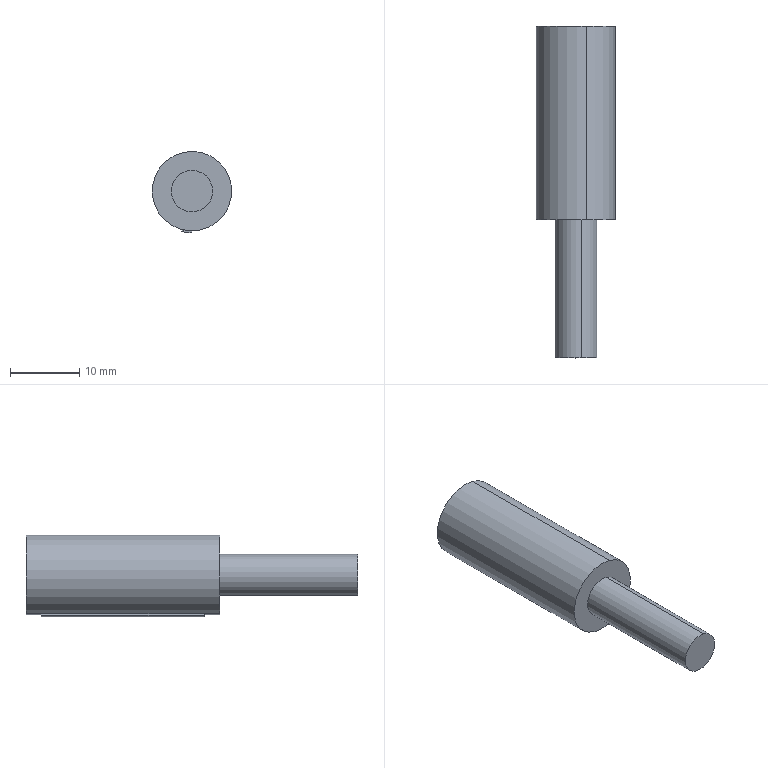Component | SolidWorks | Hinge2-1 | 1 solid | 13 faces | box 11.5 x 48 x 11.75 mm | volume 3483 mm3 | plane 9 | cylinder 4 | commonest cylinder face diameters 6 x2 11.5 x2
build123d program:
from build123d import *

# Parameters (mm, degrees)
SKETCH1_2_R              = 5.75
BOSS_EXTRUDE1_DEPTH      = 14
BOSS_EXTRUDE2_REACH      = 23.728
BOSS_EXTRUDE2_END_RADIUS = 5.75
SKETCH2_W                = 1.461
SKETCH2_H                = 23.562
SKETCH3_R                = 3
BOSS_EXTRUDE3_DEPTH      = 20
CUT_EXTRUDE1_DEPTH       = 13
CUT_EXTRUDE1_DEPTH_BACK  = 13


with BuildPart() as part:
    # Sketch1_2 → Boss-Extrude1 (new, symmetric)
    with BuildSketch(Plane(origin=(0, 0, 0), x_dir=(1, 0, 0), z_dir=(0, 1, 0))):
        with Locations(Location((-6, -6, 0), (0, 0, 270))):
            Circle(SKETCH1_2_R)
    extrude(amount=BOSS_EXTRUDE1_DEPTH, both=True)

    # Boss-Extrude2: up to this cylinder (the profile starts outside it)
    boss_extrude2_end = Plane(origin=(-6, 0, 6), z_dir=(0, -1, 0)) * Cylinder(BOSS_EXTRUDE2_END_RADIUS, 59.956, mode=Mode.PRIVATE)
    # Sketch2 → Boss-Extrude2 (add, up to the surface)
    with BuildSketch(Plane.XY, mode=Mode.PRIVATE) as boss_extrude2_sk1:
        with Locations((-5.269, 0)):
            Rectangle(SKETCH2_W, SKETCH2_H)
    boss_extrude2_tool1 = extrude(boss_extrude2_sk1.sketch, amount=BOSS_EXTRUDE2_REACH, mode=Mode.PRIVATE) - boss_extrude2_end
    add(boss_extrude2_tool1.solids().sort_by_distance((-5.269, 0, 0))[0])

    # Sketch3 → Boss-Extrude3 (add)
    with BuildSketch(Plane.XZ.offset(14)):
        with Locations(Location((-6, 6, 0), (0, 0, 90))):
            Circle(SKETCH3_R)
    extrude(amount=BOSS_EXTRUDE3_DEPTH)

    # Sketch1 → Cut-Extrude1 (cut, two sides: drawn at the far end of the back side and taken through both)
    with BuildSketch(Plane(origin=(0, 0, 0), x_dir=(1, 0, 0), z_dir=(0, 1, 0)).offset(-CUT_EXTRUDE1_DEPTH_BACK)):
        Polygon((-7.5, 0.6087), (-3, -0.5914), (-3, 2), (-7.5, 2), align=None)
    extrude(amount=CUT_EXTRUDE1_DEPTH + CUT_EXTRUDE1_DEPTH_BACK, mode=Mode.SUBTRACT)


solid = part.part

# Placed as in the assembly
solid = solid.moved(Location((227.642, -308.131, 905.044), (0, 14.933, 0)))
STEP:
#1=CARTESIAN_POINT('',(8.764,-13.47,35.807));
#2=VERTEX_POINT('',#1);
#3=CARTESIAN_POINT('',(8.825,-13.47,36.035));
#4=VERTEX_POINT('',#3);
#5=CARTESIAN_POINT('',(8.795,-13.47,35.921));
#6=DIRECTION('',(0.,-1.,0.));
#7=DIRECTION('',(-0.2577,0.,-0.9662));
#8=AXIS2_PLACEMENT_3D('',#5,#6,#7);
#9=CIRCLE('',#8,0.1181);
#10=EDGE_CURVE('',#2,#4,#9,.T.);
#11=ORIENTED_EDGE('',*,*,#10,.F.);
#12=CARTESIAN_POINT('',(8.764,-12.682,35.807));
#13=VERTEX_POINT('',#12);
#14=CARTESIAN_POINT('',(8.764,-13.47,35.807));
#15=DIRECTION('',(0.,1.,0.));
#16=VECTOR('',#15,39.37);
#17=LINE('',#14,#16);
#18=EDGE_CURVE('',#2,#13,#17,.T.);
#19=ORIENTED_EDGE('',*,*,#18,.T.);
#20=CARTESIAN_POINT('',(8.825,-12.682,36.035));
#21=VERTEX_POINT('',#20);
#22=CARTESIAN_POINT('',(8.795,-12.682,35.921));
#23=DIRECTION('',(0.,-1.,0.));
#24=DIRECTION('',(0.2577,0.,0.9662));
#25=AXIS2_PLACEMENT_3D('',#22,#23,#24);
#26=CIRCLE('',#25,0.1181);
#27=EDGE_CURVE('',#13,#21,#26,.T.);
#28=ORIENTED_EDGE('',*,*,#27,.T.);
#29=CARTESIAN_POINT('',(8.825,-13.47,36.035));
#30=DIRECTION('',(0.,1.,0.));
#31=VECTOR('',#30,39.37);
#32=LINE('',#29,#31);
#33=EDGE_CURVE('',#4,#21,#32,.T.);
#34=ORIENTED_EDGE('',*,*,#33,.F.);
#35=EDGE_LOOP('',(#11,#19,#28,#34));
#36=FACE_OUTER_BOUND('',#35,.T.);
#37=CARTESIAN_POINT('',(8.795,-13.47,35.921));
#38=DIRECTION('',(0.,1.,0.));
#39=DIRECTION('',(0.2577,0.,0.9662));
#40=AXIS2_PLACEMENT_3D('',#37,#38,#39);
#41=CYLINDRICAL_SURFACE('',#40,0.1181);
#42=ADVANCED_FACE('',(#36),#41,.T.);
#43=CARTESIAN_POINT('',(8.853,-11.58,36.139));
#44=VERTEX_POINT('',#43);
#45=CARTESIAN_POINT('',(8.737,-11.58,35.702));
#46=VERTEX_POINT('',#45);
#47=CARTESIAN_POINT('',(8.795,-11.58,35.921));
#48=DIRECTION('',(0.,1.,0.));
#49=DIRECTION('',(0.2577,0.,0.9662));
#50=AXIS2_PLACEMENT_3D('',#47,#48,#49);
#51=CIRCLE('',#50,0.2264);
#52=EDGE_CURVE('',#44,#46,#51,.T.);
#53=ORIENTED_EDGE('',*,*,#52,.F.);
#54=CARTESIAN_POINT('',(8.853,-12.682,36.139));
#55=VERTEX_POINT('',#54);
#56=CARTESIAN_POINT('',(8.853,-11.58,36.139));
#57=DIRECTION('',(0.,-1.,0.));
#58=VECTOR('',#57,39.37);
#59=LINE('',#56,#58);
#60=EDGE_CURVE('',#44,#55,#59,.T.);
#61=ORIENTED_EDGE('',*,*,#60,.T.);
#62=CARTESIAN_POINT('',(8.737,-12.682,35.702));
#63=VERTEX_POINT('',#62);
#64=CARTESIAN_POINT('',(8.795,-12.682,35.921));
#65=DIRECTION('',(0.,1.,0.));
#66=DIRECTION('',(0.2577,0.,0.9662));
#67=AXIS2_PLACEMENT_3D('',#64,#65,#66);
#68=CIRCLE('',#67,0.2264);
#69=EDGE_CURVE('',#55,#63,#68,.T.);
#70=ORIENTED_EDGE('',*,*,#69,.T.);
#71=CARTESIAN_POINT('',(8.737,-12.595,35.702));
#72=VERTEX_POINT('',#71);
#73=CARTESIAN_POINT('',(8.737,-11.58,35.702));
#74=DIRECTION('',(0.,-1.,0.));
#75=VECTOR('',#74,39.37);
#76=LINE('',#73,#75);
#77=EDGE_CURVE('',#72,#63,#76,.T.);
#78=ORIENTED_EDGE('',*,*,#77,.F.);
#79=CARTESIAN_POINT('',(8.794,-12.595,35.694));
#80=VERTEX_POINT('',#79);
#81=CARTESIAN_POINT('',(8.795,-12.595,35.921));
#82=DIRECTION('',(0.,-1.,0.));
#83=DIRECTION('',(0.2577,0.,0.9662));
#84=AXIS2_PLACEMENT_3D('',#81,#82,#83);
#85=CIRCLE('',#84,0.2264);
#86=EDGE_CURVE('',#72,#80,#85,.T.);
#87=ORIENTED_EDGE('',*,*,#86,.T.);
#88=CARTESIAN_POINT('',(8.794,-11.667,35.694));
#89=VERTEX_POINT('',#88);
#90=CARTESIAN_POINT('',(8.794,-11.58,35.694));
#91=DIRECTION('',(0.,1.,0.));
#92=VECTOR('',#91,39.37);
#93=LINE('',#90,#92);
#94=EDGE_CURVE('',#80,#89,#93,.T.);
#95=ORIENTED_EDGE('',*,*,#94,.T.);
#96=CARTESIAN_POINT('',(8.737,-11.667,35.702));
#97=VERTEX_POINT('',#96);
#98=CARTESIAN_POINT('',(8.795,-11.667,35.921));
#99=DIRECTION('',(0.,1.,0.));
#100=DIRECTION('',(-0.2577,0.,-0.9662));
#101=AXIS2_PLACEMENT_3D('',#98,#99,#100);
#102=CIRCLE('',#101,0.2264);
#103=EDGE_CURVE('',#89,#97,#102,.T.);
#104=ORIENTED_EDGE('',*,*,#103,.T.);
#105=CARTESIAN_POINT('',(8.737,-11.58,35.702));
#106=DIRECTION('',(0.,-1.,0.));
#107=VECTOR('',#106,39.37);
#108=LINE('',#105,#107);
#109=EDGE_CURVE('',#46,#97,#108,.T.);
#110=ORIENTED_EDGE('',*,*,#109,.F.);
#111=EDGE_LOOP('',(#53,#61,#70,#78,#87,#95,#104,#110));
#112=FACE_OUTER_BOUND('',#111,.T.);
#113=CARTESIAN_POINT('',(8.795,-11.58,35.921));
#114=DIRECTION('',(0.,-1.,0.));
#115=DIRECTION('',(-0.2577,0.,-0.9662));
#116=AXIS2_PLACEMENT_3D('',#113,#114,#115);
#117=CYLINDRICAL_SURFACE('',#116,0.2264);
#118=ADVANCED_FACE('',(#112),#117,.T.);
#119=CARTESIAN_POINT('',(8.791,-12.595,35.685));
#120=VERTEX_POINT('',#119);
#121=CARTESIAN_POINT('',(8.764,-12.595,35.685));
#122=VERTEX_POINT('',#121);
#123=CARTESIAN_POINT('',(5081.383,-12.595,35.685));
#124=DIRECTION('',(-1.,0.,-0.));
#125=VECTOR('',#124,39.37);
#126=LINE('',#123,#125);
#127=EDGE_CURVE('',#120,#122,#126,.T.);
#128=ORIENTED_EDGE('',*,*,#127,.F.);
#129=CARTESIAN_POINT('',(5081.383,-12.595,19055.919));
#130=DIRECTION('',(-0.2577,0.,-0.9662));
#131=VECTOR('',#130,39.37);
#132=LINE('',#129,#131);
#133=EDGE_CURVE('',#80,#120,#132,.T.);
#134=ORIENTED_EDGE('',*,*,#133,.F.);
#135=ORIENTED_EDGE('',*,*,#86,.F.);
#136=CARTESIAN_POINT('',(8.734,-12.595,35.693));
#137=VERTEX_POINT('',#136);
#138=CARTESIAN_POINT('',(5081.327,-12.595,19055.934));
#139=DIRECTION('',(-0.2577,0.,-0.9662));
#140=VECTOR('',#139,39.37);
#141=LINE('',#138,#140);
#142=EDGE_CURVE('',#72,#137,#141,.T.);
#143=ORIENTED_EDGE('',*,*,#142,.T.);
#144=CARTESIAN_POINT('',(8.79,-12.595,35.678));
#145=DIRECTION('',(0.9662,0.,-0.2577));
#146=VECTOR('',#145,39.37);
#147=LINE('',#144,#146);
#148=EDGE_CURVE('',#137,#122,#147,.T.);
#149=ORIENTED_EDGE('',*,*,#148,.T.);
#150=EDGE_LOOP('',(#128,#134,#135,#143,#149));
#151=FACE_OUTER_BOUND('',#150,.T.);
#152=CARTESIAN_POINT('',(5081.383,-12.595,19055.919));
#153=DIRECTION('',(0.,1.,0.));
#154=DIRECTION('',(0.2577,0.,0.9662));
#155=AXIS2_PLACEMENT_3D('',#152,#153,#154);
#156=PLANE('',#155);
#157=ADVANCED_FACE('',(#151),#156,.F.);
#158=CARTESIAN_POINT('',(8.764,-11.667,35.685));
#159=VERTEX_POINT('',#158);
#160=CARTESIAN_POINT('',(8.764,-12.131,35.685));
#161=DIRECTION('',(0.,1.,0.));
#162=VECTOR('',#161,39.37);
#163=LINE('',#160,#162);
#164=EDGE_CURVE('',#122,#159,#163,.T.);
#165=ORIENTED_EDGE('',*,*,#164,.F.);
#166=ORIENTED_EDGE('',*,*,#148,.F.);
#167=CARTESIAN_POINT('',(8.734,-11.667,35.693));
#168=VERTEX_POINT('',#167);
#169=CARTESIAN_POINT('',(8.734,-12.595,35.693));
#170=DIRECTION('',(0.,-1.,0.));
#171=VECTOR('',#170,39.37);
#172=LINE('',#169,#171);
#173=EDGE_CURVE('',#168,#137,#172,.T.);
#174=ORIENTED_EDGE('',*,*,#173,.F.);
#175=CARTESIAN_POINT('',(8.79,-11.667,35.678));
#176=DIRECTION('',(-0.9662,0.,0.2577));
#177=VECTOR('',#176,39.37);
#178=LINE('',#175,#177);
#179=EDGE_CURVE('',#159,#168,#178,.T.);
#180=ORIENTED_EDGE('',*,*,#179,.F.);
#181=EDGE_LOOP('',(#165,#166,#174,#180));
#182=FACE_OUTER_BOUND('',#181,.T.);
#183=CARTESIAN_POINT('',(8.962,-12.131,35.632));
#184=DIRECTION('',(0.2577,0.,0.9662));
#185=DIRECTION('',(0.9662,0.,-0.2577));
#186=AXIS2_PLACEMENT_3D('',#183,#184,#185);
#187=PLANE('',#186);
#188=ADVANCED_FACE('',(#182),#187,.F.);
#189=CARTESIAN_POINT('',(8.791,-11.667,35.685));
#190=VERTEX_POINT('',#189);
#191=CARTESIAN_POINT('',(8.791,-12.595,35.685));
#192=DIRECTION('',(0.,-1.,0.));
#193=VECTOR('',#192,39.37);
#194=LINE('',#191,#193);
#195=EDGE_CURVE('',#190,#120,#194,.T.);
#196=ORIENTED_EDGE('',*,*,#195,.F.);
#197=CARTESIAN_POINT('',(5081.383,-11.667,19055.919));
#198=DIRECTION('',(-0.2577,0.,-0.9662));
#199=VECTOR('',#198,39.37);
#200=LINE('',#197,#199);
#201=EDGE_CURVE('',#89,#190,#200,.T.);
#202=ORIENTED_EDGE('',*,*,#201,.F.);
#203=ORIENTED_EDGE('',*,*,#94,.F.);
#204=ORIENTED_EDGE('',*,*,#133,.T.);
#205=EDGE_LOOP('',(#196,#202,#203,#204));
#206=FACE_OUTER_BOUND('',#205,.T.);
#207=CARTESIAN_POINT('',(5081.383,-12.595,19055.919));
#208=DIRECTION('',(-0.9662,0.,0.2577));
#209=DIRECTION('',(0.2577,0.,0.9662));
#210=AXIS2_PLACEMENT_3D('',#207,#208,#209);
#211=PLANE('',#210);
#212=ADVANCED_FACE('',(#206),#211,.F.);
#213=CARTESIAN_POINT('',(5081.383,-11.667,35.685));
#214=DIRECTION('',(1.,0.,0.));
#215=VECTOR('',#214,39.37);
#216=LINE('',#213,#215);
#217=EDGE_CURVE('',#159,#190,#216,.T.);
#218=ORIENTED_EDGE('',*,*,#217,.F.);
#219=ORIENTED_EDGE('',*,*,#179,.T.);
#220=CARTESIAN_POINT('',(5081.327,-11.667,19055.934));
#221=DIRECTION('',(-0.2577,0.,-0.9662));
#222=VECTOR('',#221,39.37);
#223=LINE('',#220,#222);
#224=EDGE_CURVE('',#97,#168,#223,.T.);
#225=ORIENTED_EDGE('',*,*,#224,.F.);
#226=ORIENTED_EDGE('',*,*,#103,.F.);
#227=ORIENTED_EDGE('',*,*,#201,.T.);
#228=EDGE_LOOP('',(#218,#219,#225,#226,#227));
#229=FACE_OUTER_BOUND('',#228,.T.);
#230=CARTESIAN_POINT('',(5081.383,-11.667,19055.919));
#231=DIRECTION('',(0.,-1.,0.));
#232=DIRECTION('',(-0.2577,0.,-0.9662));
#233=AXIS2_PLACEMENT_3D('',#230,#231,#232);
#234=PLANE('',#233);
#235=ADVANCED_FACE('',(#229),#234,.F.);
#236=CARTESIAN_POINT('',(8.795,-12.682,35.921));
#237=DIRECTION('',(0.,1.,0.));
#238=DIRECTION('',(0.2577,0.,0.9662));
#239=AXIS2_PLACEMENT_3D('',#236,#237,#238);
#240=CIRCLE('',#239,0.2264);
#241=EDGE_CURVE('',#63,#55,#240,.T.);
#242=ORIENTED_EDGE('',*,*,#241,.F.);
#243=ORIENTED_EDGE('',*,*,#69,.F.);
#244=EDGE_LOOP('',(#242,#243));
#245=FACE_OUTER_BOUND('',#244,.T.);
#246=CARTESIAN_POINT('',(8.795,-12.682,35.921));
#247=DIRECTION('',(0.,-1.,0.));
#248=DIRECTION('',(0.2577,0.,0.9662));
#249=AXIS2_PLACEMENT_3D('',#246,#247,#248);
#250=CIRCLE('',#249,0.1181);
#251=EDGE_CURVE('',#21,#13,#250,.T.);
#252=ORIENTED_EDGE('',*,*,#251,.F.);
#253=ORIENTED_EDGE('',*,*,#27,.F.);
#254=EDGE_LOOP('',(#252,#253));
#255=FACE_BOUND('',#254,.T.);
#256=CARTESIAN_POINT('',(8.795,-12.682,35.921));
#257=DIRECTION('',(0.,1.,0.));
#258=DIRECTION('',(0.2577,0.,0.9662));
#259=AXIS2_PLACEMENT_3D('',#256,#257,#258);
#260=PLANE('',#259);
#261=ADVANCED_FACE('',(#245,#255),#260,.F.);
#262=ORIENTED_EDGE('',*,*,#60,.F.);
#263=CARTESIAN_POINT('',(8.795,-11.58,35.921));
#264=DIRECTION('',(0.,1.,0.));
#265=DIRECTION('',(0.2577,0.,0.9662));
#266=AXIS2_PLACEMENT_3D('',#263,#264,#265);
#267=CIRCLE('',#266,0.2264);
#268=EDGE_CURVE('',#46,#44,#267,.T.);
#269=ORIENTED_EDGE('',*,*,#268,.F.);
#270=ORIENTED_EDGE('',*,*,#109,.T.);
#271=CARTESIAN_POINT('',(8.737,-11.58,35.702));
#272=DIRECTION('',(0.,-1.,0.));
#273=VECTOR('',#272,39.37);
#274=LINE('',#271,#273);
#275=EDGE_CURVE('',#97,#72,#274,.T.);
#276=ORIENTED_EDGE('',*,*,#275,.T.);
#277=ORIENTED_EDGE('',*,*,#77,.T.);
#278=ORIENTED_EDGE('',*,*,#241,.T.);
#279=EDGE_LOOP('',(#262,#269,#270,#276,#277,#278));
#280=FACE_OUTER_BOUND('',#279,.T.);
#281=CARTESIAN_POINT('',(8.795,-11.58,35.921));
#282=DIRECTION('',(0.,-1.,0.));
#283=DIRECTION('',(-0.2577,0.,-0.9662));
#284=AXIS2_PLACEMENT_3D('',#281,#282,#283);
#285=CYLINDRICAL_SURFACE('',#284,0.2264);
#286=ADVANCED_FACE('',(#280),#285,.T.);
#287=ORIENTED_EDGE('',*,*,#268,.T.);
#288=ORIENTED_EDGE('',*,*,#52,.T.);
#289=EDGE_LOOP('',(#287,#288));
#290=FACE_OUTER_BOUND('',#289,.T.);
#291=CARTESIAN_POINT('',(8.795,-11.58,35.921));
#292=DIRECTION('',(0.,1.,0.));
#293=DIRECTION('',(0.2577,0.,0.9662));
#294=AXIS2_PLACEMENT_3D('',#291,#292,#293);
#295=PLANE('',#294);
#296=ADVANCED_FACE('',(#290),#295,.T.);
#297=ORIENTED_EDGE('',*,*,#275,.F.);
#298=ORIENTED_EDGE('',*,*,#224,.T.);
#299=ORIENTED_EDGE('',*,*,#173,.T.);
#300=ORIENTED_EDGE('',*,*,#142,.F.);
#301=EDGE_LOOP('',(#297,#298,#299,#300));
#302=FACE_OUTER_BOUND('',#301,.T.);
#303=CARTESIAN_POINT('',(5081.327,-12.595,19055.934));
#304=DIRECTION('',(0.9662,0.,-0.2577));
#305=DIRECTION('',(-0.2577,0.,-0.9662));
#306=AXIS2_PLACEMENT_3D('',#303,#304,#305);
#307=PLANE('',#306);
#308=ADVANCED_FACE('',(#302),#307,.F.);
#309=ORIENTED_EDGE('',*,*,#18,.F.);
#310=CARTESIAN_POINT('',(8.795,-13.47,35.921));
#311=DIRECTION('',(0.,-1.,0.));
#312=DIRECTION('',(-0.2577,0.,-0.9662));
#313=AXIS2_PLACEMENT_3D('',#310,#311,#312);
#314=CIRCLE('',#313,0.1181);
#315=EDGE_CURVE('',#4,#2,#314,.T.);
#316=ORIENTED_EDGE('',*,*,#315,.F.);
#317=ORIENTED_EDGE('',*,*,#33,.T.);
#318=ORIENTED_EDGE('',*,*,#251,.T.);
#319=EDGE_LOOP('',(#309,#316,#317,#318));
#320=FACE_OUTER_BOUND('',#319,.T.);
#321=CARTESIAN_POINT('',(8.795,-13.47,35.921));
#322=DIRECTION('',(0.,1.,0.));
#323=DIRECTION('',(0.2577,0.,0.9662));
#324=AXIS2_PLACEMENT_3D('',#321,#322,#323);
#325=CYLINDRICAL_SURFACE('',#324,0.1181);
#326=ADVANCED_FACE('',(#320),#325,.T.);
#327=ORIENTED_EDGE('',*,*,#315,.T.);
#328=ORIENTED_EDGE('',*,*,#10,.T.);
#329=EDGE_LOOP('',(#327,#328));
#330=FACE_OUTER_BOUND('',#329,.T.);
#331=CARTESIAN_POINT('',(8.795,-13.47,35.921));
#332=DIRECTION('',(0.,-1.,0.));
#333=DIRECTION('',(-0.2577,0.,-0.9662));
#334=AXIS2_PLACEMENT_3D('',#331,#332,#333);
#335=PLANE('',#334);
#336=ADVANCED_FACE('',(#330),#335,.T.);
#337=ORIENTED_EDGE('',*,*,#127,.T.);
#338=ORIENTED_EDGE('',*,*,#164,.T.);
#339=ORIENTED_EDGE('',*,*,#217,.T.);
#340=ORIENTED_EDGE('',*,*,#195,.T.);
#341=EDGE_LOOP('',(#337,#338,#339,#340));
#342=FACE_OUTER_BOUND('',#341,.T.);
#343=CARTESIAN_POINT('',(8.671,-11.619,35.685));
#344=DIRECTION('',(0.,0.,-1.));
#345=DIRECTION('',(-1.,0.,-0.));
#346=AXIS2_PLACEMENT_3D('',#343,#344,#345);
#347=PLANE('',#346);
#348=ADVANCED_FACE('',(#342),#347,.T.);
#349=CLOSED_SHELL('',(#42,#118,#157,#188,#212,#235,#261,#286,#296,#308,#326,#336,#348));
#350=MANIFOLD_SOLID_BREP('',#349);
#351=CARTESIAN_POINT('',(0.,0.,0.));
#352=DIRECTION('',(0.,0.,1.));
#353=DIRECTION('',(1.,0.,0.));
#354=AXIS2_PLACEMENT_3D('',#351,#352,#353);
#355=(LENGTH_UNIT()NAMED_UNIT(*)SI_UNIT($,.METRE.));
#356=LENGTH_MEASURE_WITH_UNIT(LENGTH_MEASURE(0.0254),#355);
#357=DIMENSIONAL_EXPONENTS(1.,0.,0.,0.,0.,0.,0.);
#358=(CONVERSION_BASED_UNIT('',#356)LENGTH_UNIT()NAMED_UNIT(#357));
#359=UNCERTAINTY_MEASURE_WITH_UNIT(LENGTH_MEASURE(0.00001),#358,'','');
#360=(NAMED_UNIT(*)PLANE_ANGLE_UNIT()SI_UNIT($,.RADIAN.));
#361=(NAMED_UNIT(*)SI_UNIT($,.STERADIAN.)SOLID_ANGLE_UNIT());
#362=(GEOMETRIC_REPRESENTATION_CONTEXT(3)GLOBAL_UNCERTAINTY_ASSIGNED_CONTEXT((#359))GLOBAL_UNIT_ASSIGNED_CONTEXT((#358,#360,#361))REPRESENTATION_CONTEXT('',''));
#363=ADVANCED_BREP_SHAPE_REPRESENTATION('',(#350,#354),#362);
#364=COLOUR_RGB('',0.7922,0.8196,0.9333);
#365=FILL_AREA_STYLE_COLOUR('',#364);
#366=FILL_AREA_STYLE('',(#365));
#367=SURFACE_STYLE_FILL_AREA(#366);
#368=SURFACE_SIDE_STYLE('',(#367));
#369=SURFACE_STYLE_USAGE(.BOTH.,#368);
#370=PRESENTATION_STYLE_ASSIGNMENT((#369));
#371=STYLED_ITEM('',(#370),#350);
#372=PRESENTATION_LAYER_ASSIGNMENT('','',(#371));
#373=(LENGTH_UNIT()NAMED_UNIT(*)SI_UNIT($,.METRE.));
#374=LENGTH_MEASURE_WITH_UNIT(LENGTH_MEASURE(0.0254),#373);
#375=DIMENSIONAL_EXPONENTS(1.,0.,0.,0.,0.,0.,0.);
#376=(CONVERSION_BASED_UNIT('',#374)LENGTH_UNIT()NAMED_UNIT(#375));
#377=UNCERTAINTY_MEASURE_WITH_UNIT(LENGTH_MEASURE(0.00001),#376,'','');
#378=(NAMED_UNIT(*)PLANE_ANGLE_UNIT()SI_UNIT($,.RADIAN.));
#379=(NAMED_UNIT(*)SI_UNIT($,.STERADIAN.)SOLID_ANGLE_UNIT());
#380=(GEOMETRIC_REPRESENTATION_CONTEXT(3)GLOBAL_UNCERTAINTY_ASSIGNED_CONTEXT((#377))GLOBAL_UNIT_ASSIGNED_CONTEXT((#376,#378,#379))REPRESENTATION_CONTEXT('',''));
#381=MECHANICAL_DESIGN_GEOMETRIC_PRESENTATION_REPRESENTATION('',(#371),#380);